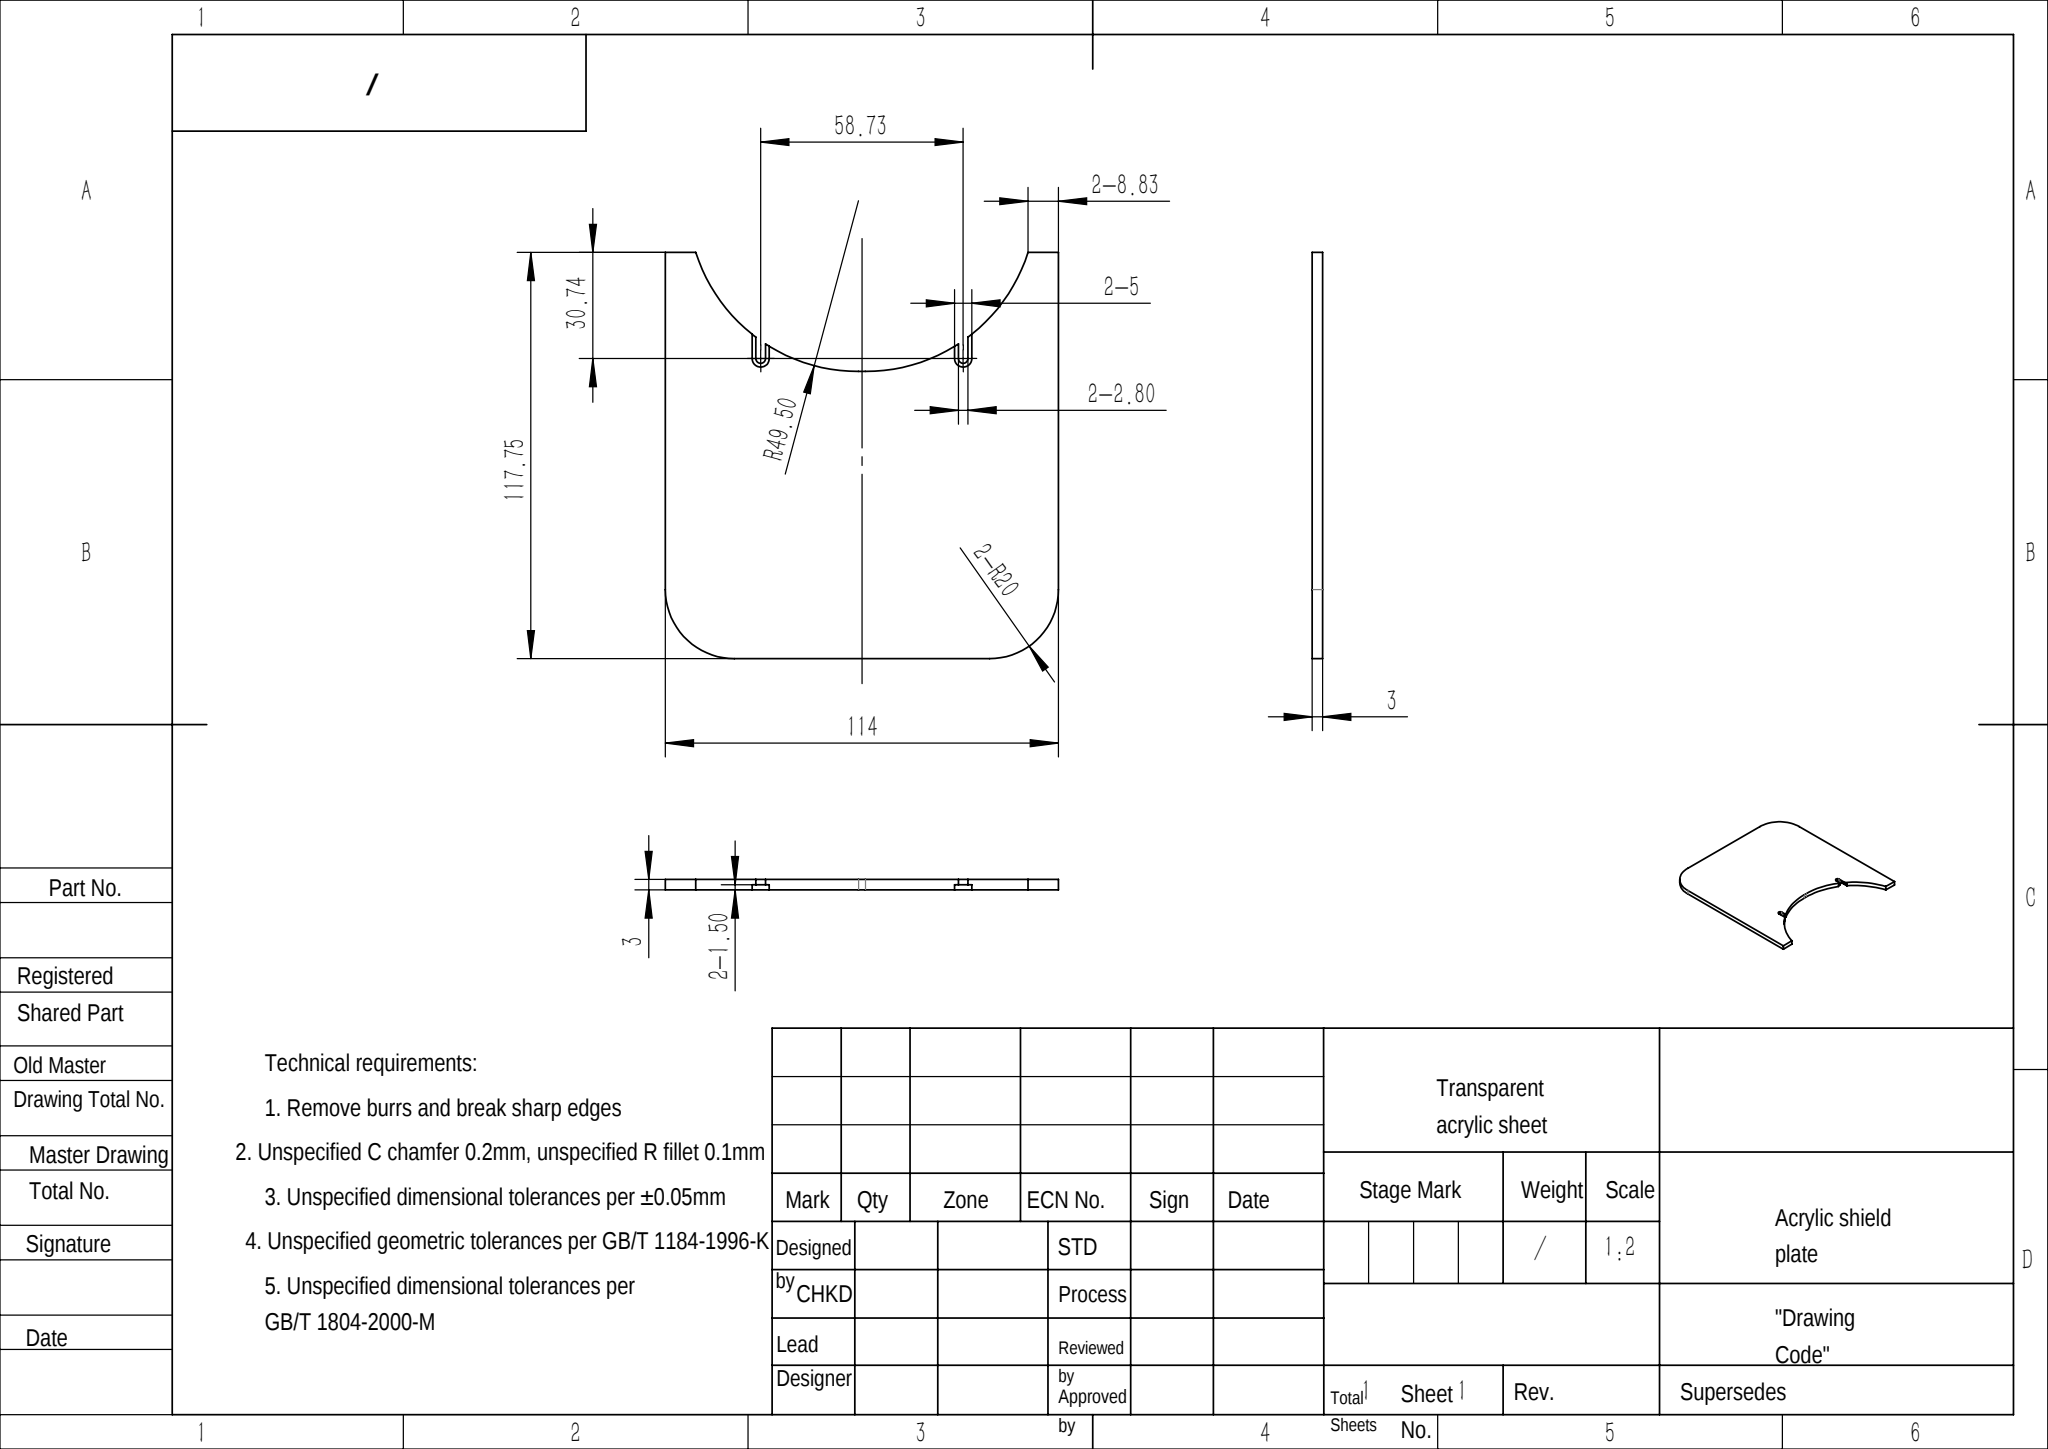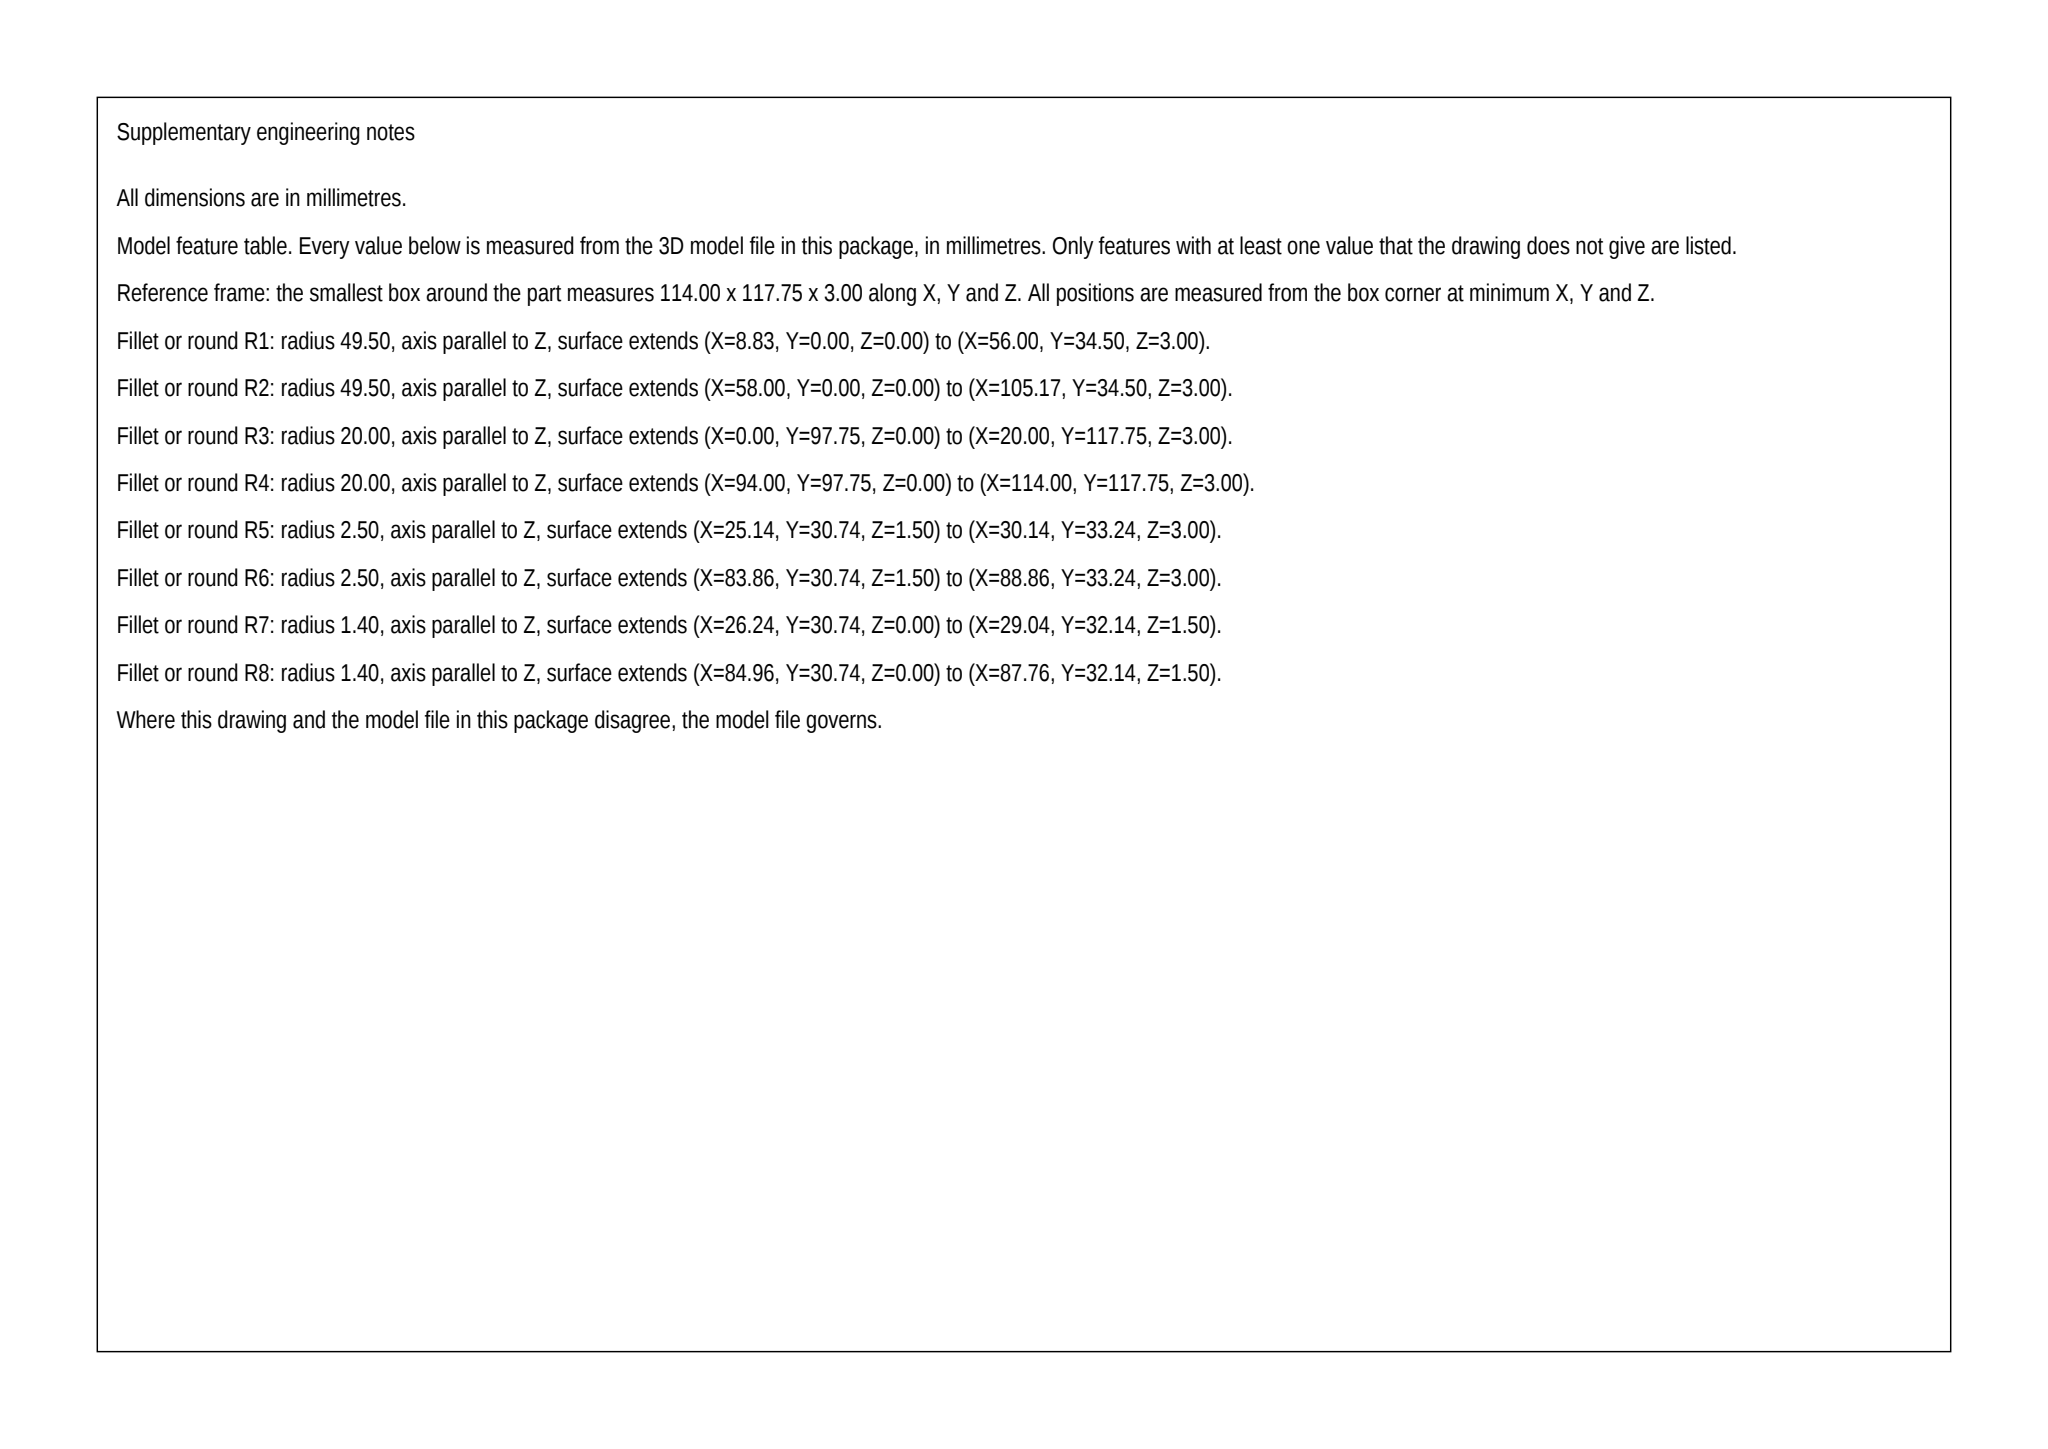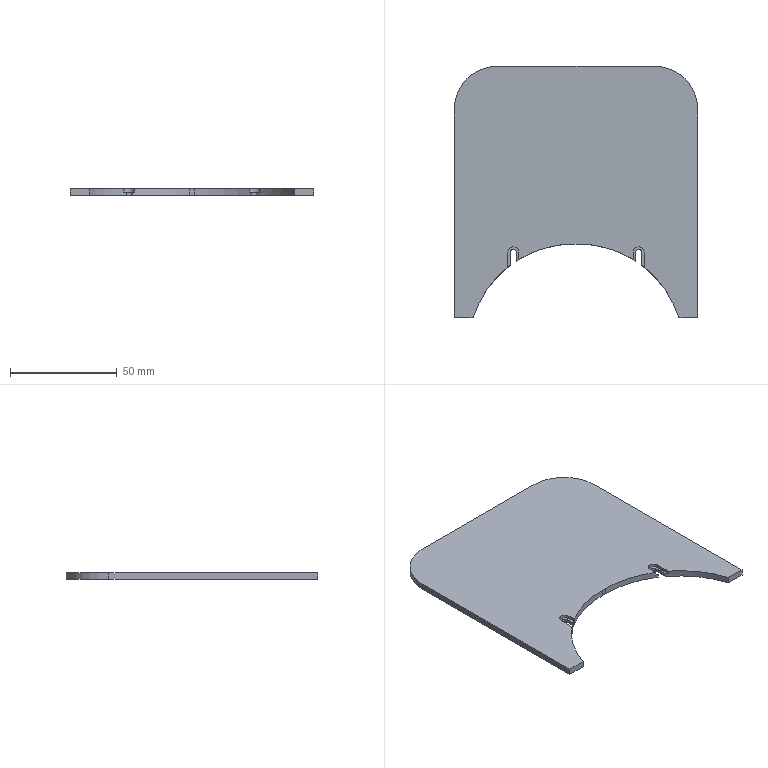Part | SolidWorks | mm | material Transparent acrylic sheet | 1 solid | 28 faces | box 114 x 117.75 x 3 mm | volume 32227 mm3 | plane 18 | cylinder 10 | commonest cylinder face diameters 99 x4 2.8 x2 40 x2 5 x2
STEP:
#1=CARTESIAN_POINT('',(27.964,141.858,1.5));
#2=VERTEX_POINT('',#1);
#3=CARTESIAN_POINT('',(30.764,141.858,1.5));
#4=VERTEX_POINT('',#3);
#5=CARTESIAN_POINT('',(29.364,141.858,1.5));
#6=DIRECTION('',(0.,0.,-1.));
#7=DIRECTION('',(1.,0.,0.));
#8=AXIS2_PLACEMENT_3D('',#5,#6,#7);
#9=CIRCLE('',#8,1.4);
#10=EDGE_CURVE('',#2,#4,#9,.T.);
#11=ORIENTED_EDGE('',*,*,#10,.F.);
#12=CARTESIAN_POINT('',(27.964,141.858,0.));
#13=VERTEX_POINT('',#12);
#14=CARTESIAN_POINT('',(27.964,141.858,-7.));
#15=DIRECTION('',(0.,0.,1.));
#16=VECTOR('',#15,1000.);
#17=LINE('',#14,#16);
#18=EDGE_CURVE('',#13,#2,#17,.T.);
#19=ORIENTED_EDGE('',*,*,#18,.F.);
#20=CARTESIAN_POINT('',(30.764,141.858,0.));
#21=VERTEX_POINT('',#20);
#22=CARTESIAN_POINT('',(29.364,141.858,0.));
#23=DIRECTION('',(0.,0.,1.));
#24=DIRECTION('',(1.,0.,0.));
#25=AXIS2_PLACEMENT_3D('',#22,#23,#24);
#26=CIRCLE('',#25,1.4);
#27=EDGE_CURVE('',#21,#13,#26,.T.);
#28=ORIENTED_EDGE('',*,*,#27,.F.);
#29=CARTESIAN_POINT('',(30.764,141.858,-7.));
#30=DIRECTION('',(0.,0.,1.));
#31=VECTOR('',#30,1000.);
#32=LINE('',#29,#31);
#33=EDGE_CURVE('',#21,#4,#32,.T.);
#34=ORIENTED_EDGE('',*,*,#33,.T.);
#35=EDGE_LOOP('',(#11,#19,#28,#34));
#36=FACE_OUTER_BOUND('',#35,.T.);
#37=CARTESIAN_POINT('',(29.364,141.858,-7.));
#38=DIRECTION('',(0.,0.,1.));
#39=DIRECTION('',(1.,0.,0.));
#40=AXIS2_PLACEMENT_3D('',#37,#38,#39);
#41=CYLINDRICAL_SURFACE('',#40,1.4);
#42=ADVANCED_FACE('',(#36),#41,.F.);
#43=CARTESIAN_POINT('',(30.764,135.668,1.5));
#44=VERTEX_POINT('',#43);
#45=CARTESIAN_POINT('',(30.764,132.725,1.5));
#46=DIRECTION('',(0.,-1.,0.));
#47=VECTOR('',#46,1000.);
#48=LINE('',#45,#47);
#49=EDGE_CURVE('',#4,#44,#48,.T.);
#50=ORIENTED_EDGE('',*,*,#49,.F.);
#51=ORIENTED_EDGE('',*,*,#33,.F.);
#52=CARTESIAN_POINT('',(30.764,135.668,0.));
#53=VERTEX_POINT('',#52);
#54=CARTESIAN_POINT('',(30.764,96.116,0.));
#55=DIRECTION('',(0.,1.,0.));
#56=VECTOR('',#55,1000.);
#57=LINE('',#54,#56);
#58=EDGE_CURVE('',#53,#21,#57,.T.);
#59=ORIENTED_EDGE('',*,*,#58,.F.);
#60=CARTESIAN_POINT('',(30.764,135.668,3.));
#61=DIRECTION('',(0.,0.,1.));
#62=VECTOR('',#61,1000.);
#63=LINE('',#60,#62);
#64=EDGE_CURVE('',#53,#44,#63,.T.);
#65=ORIENTED_EDGE('',*,*,#64,.T.);
#66=EDGE_LOOP('',(#50,#51,#59,#65));
#67=FACE_OUTER_BOUND('',#66,.T.);
#68=CARTESIAN_POINT('',(30.764,132.725,-7.));
#69=DIRECTION('',(1.,0.,0.));
#70=DIRECTION('',(0.,0.,-1.));
#71=AXIS2_PLACEMENT_3D('',#68,#69,#70);
#72=PLANE('',#71);
#73=ADVANCED_FACE('',(#67),#72,.F.);
#74=CARTESIAN_POINT('',(27.964,137.627,1.5));
#75=VERTEX_POINT('',#74);
#76=CARTESIAN_POINT('',(27.964,141.858,1.5));
#77=DIRECTION('',(0.,1.,0.));
#78=VECTOR('',#77,1000.);
#79=LINE('',#76,#78);
#80=EDGE_CURVE('',#75,#2,#79,.T.);
#81=ORIENTED_EDGE('',*,*,#80,.F.);
#82=CARTESIAN_POINT('',(27.964,137.627,0.));
#83=VERTEX_POINT('',#82);
#84=CARTESIAN_POINT('',(27.964,137.627,3.));
#85=DIRECTION('',(0.,0.,-1.));
#86=VECTOR('',#85,1000.);
#87=LINE('',#84,#86);
#88=EDGE_CURVE('',#75,#83,#87,.T.);
#89=ORIENTED_EDGE('',*,*,#88,.T.);
#90=CARTESIAN_POINT('',(27.964,96.116,0.));
#91=DIRECTION('',(0.,-1.,0.));
#92=VECTOR('',#91,1000.);
#93=LINE('',#90,#92);
#94=EDGE_CURVE('',#13,#83,#93,.T.);
#95=ORIENTED_EDGE('',*,*,#94,.F.);
#96=ORIENTED_EDGE('',*,*,#18,.T.);
#97=EDGE_LOOP('',(#81,#89,#95,#96));
#98=FACE_OUTER_BOUND('',#97,.T.);
#99=CARTESIAN_POINT('',(27.964,141.858,-7.));
#100=DIRECTION('',(-1.,0.,0.));
#101=DIRECTION('',(0.,0.,1.));
#102=AXIS2_PLACEMENT_3D('',#99,#100,#101);
#103=PLANE('',#102);
#104=ADVANCED_FACE('',(#98),#103,.F.);
#105=CARTESIAN_POINT('',(-30.764,141.858,1.5));
#106=VERTEX_POINT('',#105);
#107=CARTESIAN_POINT('',(-27.964,141.858,1.5));
#108=VERTEX_POINT('',#107);
#109=CARTESIAN_POINT('',(-29.364,141.858,1.5));
#110=DIRECTION('',(0.,0.,-1.));
#111=DIRECTION('',(1.,0.,0.));
#112=AXIS2_PLACEMENT_3D('',#109,#110,#111);
#113=CIRCLE('',#112,1.4);
#114=EDGE_CURVE('',#106,#108,#113,.T.);
#115=ORIENTED_EDGE('',*,*,#114,.F.);
#116=CARTESIAN_POINT('',(-30.764,141.858,0.));
#117=VERTEX_POINT('',#116);
#118=CARTESIAN_POINT('',(-30.764,141.858,-7.));
#119=DIRECTION('',(0.,0.,1.));
#120=VECTOR('',#119,1000.);
#121=LINE('',#118,#120);
#122=EDGE_CURVE('',#117,#106,#121,.T.);
#123=ORIENTED_EDGE('',*,*,#122,.F.);
#124=CARTESIAN_POINT('',(-27.964,141.858,0.));
#125=VERTEX_POINT('',#124);
#126=CARTESIAN_POINT('',(-29.364,141.858,0.));
#127=DIRECTION('',(0.,0.,1.));
#128=DIRECTION('',(1.,0.,0.));
#129=AXIS2_PLACEMENT_3D('',#126,#127,#128);
#130=CIRCLE('',#129,1.4);
#131=EDGE_CURVE('',#125,#117,#130,.T.);
#132=ORIENTED_EDGE('',*,*,#131,.F.);
#133=CARTESIAN_POINT('',(-27.964,141.858,-7.));
#134=DIRECTION('',(0.,0.,1.));
#135=VECTOR('',#134,1000.);
#136=LINE('',#133,#135);
#137=EDGE_CURVE('',#125,#108,#136,.T.);
#138=ORIENTED_EDGE('',*,*,#137,.T.);
#139=EDGE_LOOP('',(#115,#123,#132,#138));
#140=FACE_OUTER_BOUND('',#139,.T.);
#141=CARTESIAN_POINT('',(-29.364,141.858,-7.));
#142=DIRECTION('',(0.,0.,1.));
#143=DIRECTION('',(1.,0.,0.));
#144=AXIS2_PLACEMENT_3D('',#141,#142,#143);
#145=CYLINDRICAL_SURFACE('',#144,1.4);
#146=ADVANCED_FACE('',(#140),#145,.F.);
#147=CARTESIAN_POINT('',(-27.964,137.627,1.5));
#148=VERTEX_POINT('',#147);
#149=CARTESIAN_POINT('',(-27.964,131.981,1.5));
#150=DIRECTION('',(0.,-1.,0.));
#151=VECTOR('',#150,1000.);
#152=LINE('',#149,#151);
#153=EDGE_CURVE('',#108,#148,#152,.T.);
#154=ORIENTED_EDGE('',*,*,#153,.F.);
#155=ORIENTED_EDGE('',*,*,#137,.F.);
#156=CARTESIAN_POINT('',(-27.964,137.627,0.));
#157=VERTEX_POINT('',#156);
#158=CARTESIAN_POINT('',(-27.964,96.116,0.));
#159=DIRECTION('',(0.,1.,0.));
#160=VECTOR('',#159,1000.);
#161=LINE('',#158,#160);
#162=EDGE_CURVE('',#157,#125,#161,.T.);
#163=ORIENTED_EDGE('',*,*,#162,.F.);
#164=CARTESIAN_POINT('',(-27.964,137.627,3.));
#165=DIRECTION('',(0.,0.,1.));
#166=VECTOR('',#165,1000.);
#167=LINE('',#164,#166);
#168=EDGE_CURVE('',#157,#148,#167,.T.);
#169=ORIENTED_EDGE('',*,*,#168,.T.);
#170=EDGE_LOOP('',(#154,#155,#163,#169));
#171=FACE_OUTER_BOUND('',#170,.T.);
#172=CARTESIAN_POINT('',(-27.964,131.981,-7.));
#173=DIRECTION('',(1.,0.,0.));
#174=DIRECTION('',(0.,0.,-1.));
#175=AXIS2_PLACEMENT_3D('',#172,#173,#174);
#176=PLANE('',#175);
#177=ADVANCED_FACE('',(#171),#176,.F.);
#178=CARTESIAN_POINT('',(-30.764,135.668,1.5));
#179=VERTEX_POINT('',#178);
#180=CARTESIAN_POINT('',(-30.764,141.858,1.5));
#181=DIRECTION('',(0.,1.,0.));
#182=VECTOR('',#181,1000.);
#183=LINE('',#180,#182);
#184=EDGE_CURVE('',#179,#106,#183,.T.);
#185=ORIENTED_EDGE('',*,*,#184,.F.);
#186=CARTESIAN_POINT('',(-30.764,135.668,0.));
#187=VERTEX_POINT('',#186);
#188=CARTESIAN_POINT('',(-30.764,135.668,3.));
#189=DIRECTION('',(0.,0.,-1.));
#190=VECTOR('',#189,1000.);
#191=LINE('',#188,#190);
#192=EDGE_CURVE('',#179,#187,#191,.T.);
#193=ORIENTED_EDGE('',*,*,#192,.T.);
#194=CARTESIAN_POINT('',(-30.764,96.116,0.));
#195=DIRECTION('',(0.,-1.,0.));
#196=VECTOR('',#195,1000.);
#197=LINE('',#194,#196);
#198=EDGE_CURVE('',#117,#187,#197,.T.);
#199=ORIENTED_EDGE('',*,*,#198,.F.);
#200=ORIENTED_EDGE('',*,*,#122,.T.);
#201=EDGE_LOOP('',(#185,#193,#199,#200));
#202=FACE_OUTER_BOUND('',#201,.T.);
#203=CARTESIAN_POINT('',(-30.764,141.858,-7.));
#204=DIRECTION('',(-1.,0.,0.));
#205=DIRECTION('',(0.,0.,1.));
#206=AXIS2_PLACEMENT_3D('',#203,#204,#205);
#207=PLANE('',#206);
#208=ADVANCED_FACE('',(#202),#207,.F.);
#209=CARTESIAN_POINT('',(31.864,134.816,1.5));
#210=VERTEX_POINT('',#209);
#211=CARTESIAN_POINT('',(31.864,134.816,3.));
#212=VERTEX_POINT('',#211);
#213=CARTESIAN_POINT('',(31.864,134.816,3.));
#214=DIRECTION('',(0.,0.,1.));
#215=VECTOR('',#214,1000.);
#216=LINE('',#213,#215);
#217=EDGE_CURVE('',#210,#212,#216,.T.);
#218=ORIENTED_EDGE('',*,*,#217,.F.);
#219=CARTESIAN_POINT('',(1.,96.116,1.5));
#220=DIRECTION('',(0.,0.,1.));
#221=DIRECTION('',(1.,0.,0.));
#222=AXIS2_PLACEMENT_3D('',#219,#220,#221);
#223=CIRCLE('',#222,49.5);
#224=EDGE_CURVE('',#210,#44,#223,.T.);
#225=ORIENTED_EDGE('',*,*,#224,.T.);
#226=ORIENTED_EDGE('',*,*,#64,.F.);
#227=CARTESIAN_POINT('',(48.173,111.116,0.));
#228=VERTEX_POINT('',#227);
#229=CARTESIAN_POINT('',(1.,96.116,0.));
#230=DIRECTION('',(0.,0.,1.));
#231=DIRECTION('',(1.,0.,0.));
#232=AXIS2_PLACEMENT_3D('',#229,#230,#231);
#233=CIRCLE('',#232,49.5);
#234=EDGE_CURVE('',#228,#53,#233,.T.);
#235=ORIENTED_EDGE('',*,*,#234,.F.);
#236=CARTESIAN_POINT('',(48.173,111.116,3.));
#237=VERTEX_POINT('',#236);
#238=CARTESIAN_POINT('',(48.173,111.116,3.));
#239=DIRECTION('',(0.,0.,-1.));
#240=VECTOR('',#239,1000.);
#241=LINE('',#238,#240);
#242=EDGE_CURVE('',#237,#228,#241,.T.);
#243=ORIENTED_EDGE('',*,*,#242,.F.);
#244=CARTESIAN_POINT('',(1.,96.116,3.));
#245=DIRECTION('',(0.,0.,1.));
#246=DIRECTION('',(1.,0.,0.));
#247=AXIS2_PLACEMENT_3D('',#244,#245,#246);
#248=CIRCLE('',#247,49.5);
#249=EDGE_CURVE('',#237,#212,#248,.T.);
#250=ORIENTED_EDGE('',*,*,#249,.T.);
#251=EDGE_LOOP('',(#218,#225,#226,#235,#243,#250));
#252=FACE_OUTER_BOUND('',#251,.T.);
#253=CARTESIAN_POINT('',(1.,96.116,3.));
#254=DIRECTION('',(0.,0.,-1.));
#255=DIRECTION('',(-1.,0.,0.));
#256=AXIS2_PLACEMENT_3D('',#253,#254,#255);
#257=CYLINDRICAL_SURFACE('',#256,49.5);
#258=ADVANCED_FACE('',(#252),#257,.F.);
#259=CARTESIAN_POINT('',(-26.864,138.321,1.5));
#260=VERTEX_POINT('',#259);
#261=CARTESIAN_POINT('',(-26.864,138.321,3.));
#262=VERTEX_POINT('',#261);
#263=CARTESIAN_POINT('',(-26.864,138.321,3.));
#264=DIRECTION('',(0.,0.,1.));
#265=VECTOR('',#264,1000.);
#266=LINE('',#263,#265);
#267=EDGE_CURVE('',#260,#262,#266,.T.);
#268=ORIENTED_EDGE('',*,*,#267,.F.);
#269=CARTESIAN_POINT('',(-1.,96.116,1.5));
#270=DIRECTION('',(0.,0.,1.));
#271=DIRECTION('',(1.,0.,0.));
#272=AXIS2_PLACEMENT_3D('',#269,#270,#271);
#273=CIRCLE('',#272,49.5);
#274=EDGE_CURVE('',#260,#148,#273,.T.);
#275=ORIENTED_EDGE('',*,*,#274,.T.);
#276=ORIENTED_EDGE('',*,*,#168,.F.);
#277=CARTESIAN_POINT('',(-1.,145.616,0.));
#278=VERTEX_POINT('',#277);
#279=CARTESIAN_POINT('',(-1.,96.116,0.));
#280=DIRECTION('',(0.,0.,1.));
#281=DIRECTION('',(1.,0.,0.));
#282=AXIS2_PLACEMENT_3D('',#279,#280,#281);
#283=CIRCLE('',#282,49.5);
#284=EDGE_CURVE('',#278,#157,#283,.T.);
#285=ORIENTED_EDGE('',*,*,#284,.F.);
#286=CARTESIAN_POINT('',(-1.,145.616,3.));
#287=VERTEX_POINT('',#286);
#288=CARTESIAN_POINT('',(-1.,145.616,3.));
#289=DIRECTION('',(0.,0.,-1.));
#290=VECTOR('',#289,1000.);
#291=LINE('',#288,#290);
#292=EDGE_CURVE('',#287,#278,#291,.T.);
#293=ORIENTED_EDGE('',*,*,#292,.F.);
#294=CARTESIAN_POINT('',(-1.,96.116,3.));
#295=DIRECTION('',(0.,0.,1.));
#296=DIRECTION('',(1.,0.,0.));
#297=AXIS2_PLACEMENT_3D('',#294,#295,#296);
#298=CIRCLE('',#297,49.5);
#299=EDGE_CURVE('',#287,#262,#298,.T.);
#300=ORIENTED_EDGE('',*,*,#299,.T.);
#301=EDGE_LOOP('',(#268,#275,#276,#285,#293,#300));
#302=FACE_OUTER_BOUND('',#301,.T.);
#303=CARTESIAN_POINT('',(-1.,96.116,3.));
#304=DIRECTION('',(0.,0.,-1.));
#305=DIRECTION('',(-1.,0.,0.));
#306=AXIS2_PLACEMENT_3D('',#303,#304,#305);
#307=CYLINDRICAL_SURFACE('',#306,49.5);
#308=ADVANCED_FACE('',(#302),#307,.F.);
#309=CARTESIAN_POINT('',(1.,145.616,0.));
#310=VERTEX_POINT('',#309);
#311=CARTESIAN_POINT('',(-1.,145.616,0.));
#312=DIRECTION('',(1.,0.,0.));
#313=VECTOR('',#312,1000.);
#314=LINE('',#311,#313);
#315=EDGE_CURVE('',#278,#310,#314,.T.);
#316=ORIENTED_EDGE('',*,*,#315,.T.);
#317=CARTESIAN_POINT('',(1.,145.616,3.));
#318=VERTEX_POINT('',#317);
#319=CARTESIAN_POINT('',(1.,145.616,3.));
#320=DIRECTION('',(0.,0.,-1.));
#321=VECTOR('',#320,1000.);
#322=LINE('',#319,#321);
#323=EDGE_CURVE('',#318,#310,#322,.T.);
#324=ORIENTED_EDGE('',*,*,#323,.F.);
#325=CARTESIAN_POINT('',(-1.,145.616,3.));
#326=DIRECTION('',(1.,0.,0.));
#327=VECTOR('',#326,1000.);
#328=LINE('',#325,#327);
#329=EDGE_CURVE('',#287,#318,#328,.T.);
#330=ORIENTED_EDGE('',*,*,#329,.F.);
#331=ORIENTED_EDGE('',*,*,#292,.T.);
#332=EDGE_LOOP('',(#316,#324,#330,#331));
#333=FACE_OUTER_BOUND('',#332,.T.);
#334=CARTESIAN_POINT('',(-1.,145.616,3.));
#335=DIRECTION('',(0.,1.,0.));
#336=DIRECTION('',(0.,0.,1.));
#337=AXIS2_PLACEMENT_3D('',#334,#335,#336);
#338=PLANE('',#337);
#339=ADVANCED_FACE('',(#333),#338,.F.);
#340=CARTESIAN_POINT('',(26.864,138.321,3.));
#341=VERTEX_POINT('',#340);
#342=CARTESIAN_POINT('',(26.864,138.321,1.5));
#343=VERTEX_POINT('',#342);
#344=CARTESIAN_POINT('',(26.864,138.321,3.));
#345=DIRECTION('',(0.,0.,-1.));
#346=VECTOR('',#345,1000.);
#347=LINE('',#344,#346);
#348=EDGE_CURVE('',#341,#343,#347,.T.);
#349=ORIENTED_EDGE('',*,*,#348,.F.);
#350=CARTESIAN_POINT('',(1.,96.116,3.));
#351=DIRECTION('',(0.,0.,1.));
#352=DIRECTION('',(1.,0.,0.));
#353=AXIS2_PLACEMENT_3D('',#350,#351,#352);
#354=CIRCLE('',#353,49.5);
#355=EDGE_CURVE('',#341,#318,#354,.T.);
#356=ORIENTED_EDGE('',*,*,#355,.T.);
#357=ORIENTED_EDGE('',*,*,#323,.T.);
#358=CARTESIAN_POINT('',(1.,96.116,0.));
#359=DIRECTION('',(0.,0.,1.));
#360=DIRECTION('',(1.,0.,0.));
#361=AXIS2_PLACEMENT_3D('',#358,#359,#360);
#362=CIRCLE('',#361,49.5);
#363=EDGE_CURVE('',#83,#310,#362,.T.);
#364=ORIENTED_EDGE('',*,*,#363,.F.);
#365=ORIENTED_EDGE('',*,*,#88,.F.);
#366=CARTESIAN_POINT('',(1.,96.116,1.5));
#367=DIRECTION('',(0.,0.,1.));
#368=DIRECTION('',(1.,0.,0.));
#369=AXIS2_PLACEMENT_3D('',#366,#367,#368);
#370=CIRCLE('',#369,49.5);
#371=EDGE_CURVE('',#75,#343,#370,.T.);
#372=ORIENTED_EDGE('',*,*,#371,.T.);
#373=EDGE_LOOP('',(#349,#356,#357,#364,#365,#372));
#374=FACE_OUTER_BOUND('',#373,.T.);
#375=CARTESIAN_POINT('',(1.,96.116,3.));
#376=DIRECTION('',(0.,0.,-1.));
#377=DIRECTION('',(-1.,0.,0.));
#378=AXIS2_PLACEMENT_3D('',#375,#376,#377);
#379=CYLINDRICAL_SURFACE('',#378,49.5);
#380=ADVANCED_FACE('',(#374),#379,.F.);
#381=CARTESIAN_POINT('',(57.,111.116,0.));
#382=VERTEX_POINT('',#381);
#383=CARTESIAN_POINT('',(56.,111.116,0.));
#384=DIRECTION('',(1.,0.,0.));
#385=VECTOR('',#384,1000.);
#386=LINE('',#383,#385);
#387=EDGE_CURVE('',#228,#382,#386,.T.);
#388=ORIENTED_EDGE('',*,*,#387,.T.);
#389=CARTESIAN_POINT('',(57.,111.116,3.));
#390=VERTEX_POINT('',#389);
#391=CARTESIAN_POINT('',(57.,111.116,3.));
#392=DIRECTION('',(0.,0.,-1.));
#393=VECTOR('',#392,1000.);
#394=LINE('',#391,#393);
#395=EDGE_CURVE('',#390,#382,#394,.T.);
#396=ORIENTED_EDGE('',*,*,#395,.F.);
#397=CARTESIAN_POINT('',(56.,111.116,3.));
#398=DIRECTION('',(1.,0.,0.));
#399=VECTOR('',#398,1000.);
#400=LINE('',#397,#399);
#401=EDGE_CURVE('',#237,#390,#400,.T.);
#402=ORIENTED_EDGE('',*,*,#401,.F.);
#403=ORIENTED_EDGE('',*,*,#242,.T.);
#404=EDGE_LOOP('',(#388,#396,#402,#403));
#405=FACE_OUTER_BOUND('',#404,.T.);
#406=CARTESIAN_POINT('',(56.,111.116,3.));
#407=DIRECTION('',(0.,1.,0.));
#408=DIRECTION('',(0.,0.,1.));
#409=AXIS2_PLACEMENT_3D('',#406,#407,#408);
#410=PLANE('',#409);
#411=ADVANCED_FACE('',(#405),#410,.F.);
#412=CARTESIAN_POINT('',(57.,208.864,0.));
#413=VERTEX_POINT('',#412);
#414=CARTESIAN_POINT('',(57.,96.116,0.));
#415=DIRECTION('',(-0.,1.,0.));
#416=VECTOR('',#415,1000.);
#417=LINE('',#414,#416);
#418=EDGE_CURVE('',#382,#413,#417,.T.);
#419=ORIENTED_EDGE('',*,*,#418,.T.);
#420=CARTESIAN_POINT('',(57.,208.864,3.));
#421=VERTEX_POINT('',#420);
#422=CARTESIAN_POINT('',(57.,208.864,3.));
#423=DIRECTION('',(0.,0.,1.));
#424=VECTOR('',#423,1000.);
#425=LINE('',#422,#424);
#426=EDGE_CURVE('',#413,#421,#425,.T.);
#427=ORIENTED_EDGE('',*,*,#426,.T.);
#428=CARTESIAN_POINT('',(57.,96.116,3.));
#429=DIRECTION('',(-0.,1.,0.));
#430=VECTOR('',#429,1000.);
#431=LINE('',#428,#430);
#432=EDGE_CURVE('',#390,#421,#431,.T.);
#433=ORIENTED_EDGE('',*,*,#432,.F.);
#434=ORIENTED_EDGE('',*,*,#395,.T.);
#435=EDGE_LOOP('',(#419,#427,#433,#434));
#436=FACE_OUTER_BOUND('',#435,.T.);
#437=CARTESIAN_POINT('',(57.,96.116,3.));
#438=DIRECTION('',(-1.,-0.,0.));
#439=DIRECTION('',(0.,-1.,0.));
#440=AXIS2_PLACEMENT_3D('',#437,#438,#439);
#441=PLANE('',#440);
#442=ADVANCED_FACE('',(#436),#441,.F.);
#443=CARTESIAN_POINT('',(-37.,228.864,0.));
#444=VERTEX_POINT('',#443);
#445=CARTESIAN_POINT('',(37.,228.864,0.));
#446=VERTEX_POINT('',#445);
#447=CARTESIAN_POINT('',(-60.,228.864,0.));
#448=DIRECTION('',(1.,0.,0.));
#449=VECTOR('',#448,1000.);
#450=LINE('',#447,#449);
#451=EDGE_CURVE('',#444,#446,#450,.T.);
#452=ORIENTED_EDGE('',*,*,#451,.F.);
#453=CARTESIAN_POINT('',(-37.,228.864,3.));
#454=VERTEX_POINT('',#453);
#455=CARTESIAN_POINT('',(-37.,228.864,3.));
#456=DIRECTION('',(0.,0.,1.));
#457=VECTOR('',#456,1000.);
#458=LINE('',#455,#457);
#459=EDGE_CURVE('',#444,#454,#458,.T.);
#460=ORIENTED_EDGE('',*,*,#459,.T.);
#461=CARTESIAN_POINT('',(37.,228.864,3.));
#462=VERTEX_POINT('',#461);
#463=CARTESIAN_POINT('',(-60.,228.864,3.));
#464=DIRECTION('',(1.,0.,0.));
#465=VECTOR('',#464,1000.);
#466=LINE('',#463,#465);
#467=EDGE_CURVE('',#454,#462,#466,.T.);
#468=ORIENTED_EDGE('',*,*,#467,.T.);
#469=CARTESIAN_POINT('',(37.,228.864,0.));
#470=DIRECTION('',(0.,0.,-1.));
#471=VECTOR('',#470,1000.);
#472=LINE('',#469,#471);
#473=EDGE_CURVE('',#462,#446,#472,.T.);
#474=ORIENTED_EDGE('',*,*,#473,.T.);
#475=EDGE_LOOP('',(#452,#460,#468,#474));
#476=FACE_OUTER_BOUND('',#475,.T.);
#477=CARTESIAN_POINT('',(-60.,228.864,3.));
#478=DIRECTION('',(-0.,1.,0.));
#479=DIRECTION('',(-1.,-0.,0.));
#480=AXIS2_PLACEMENT_3D('',#477,#478,#479);
#481=PLANE('',#480);
#482=ADVANCED_FACE('',(#476),#481,.T.);
#483=CARTESIAN_POINT('',(-57.,111.116,3.));
#484=VERTEX_POINT('',#483);
#485=CARTESIAN_POINT('',(-57.,208.864,3.));
#486=VERTEX_POINT('',#485);
#487=CARTESIAN_POINT('',(-57.,96.116,3.));
#488=DIRECTION('',(0.,1.,0.));
#489=VECTOR('',#488,1000.);
#490=LINE('',#487,#489);
#491=EDGE_CURVE('',#484,#486,#490,.T.);
#492=ORIENTED_EDGE('',*,*,#491,.T.);
#493=CARTESIAN_POINT('',(-57.,208.864,0.));
#494=VERTEX_POINT('',#493);
#495=CARTESIAN_POINT('',(-57.,208.864,3.));
#496=DIRECTION('',(0.,0.,-1.));
#497=VECTOR('',#496,1000.);
#498=LINE('',#495,#497);
#499=EDGE_CURVE('',#486,#494,#498,.T.);
#500=ORIENTED_EDGE('',*,*,#499,.T.);
#501=CARTESIAN_POINT('',(-57.,111.116,0.));
#502=VERTEX_POINT('',#501);
#503=CARTESIAN_POINT('',(-57.,96.116,0.));
#504=DIRECTION('',(0.,1.,0.));
#505=VECTOR('',#504,1000.);
#506=LINE('',#503,#505);
#507=EDGE_CURVE('',#502,#494,#506,.T.);
#508=ORIENTED_EDGE('',*,*,#507,.F.);
#509=CARTESIAN_POINT('',(-57.,111.116,3.));
#510=DIRECTION('',(0.,0.,-1.));
#511=VECTOR('',#510,1000.);
#512=LINE('',#509,#511);
#513=EDGE_CURVE('',#484,#502,#512,.T.);
#514=ORIENTED_EDGE('',*,*,#513,.F.);
#515=EDGE_LOOP('',(#492,#500,#508,#514));
#516=FACE_OUTER_BOUND('',#515,.T.);
#517=CARTESIAN_POINT('',(-57.,96.116,3.));
#518=DIRECTION('',(-1.,0.,0.));
#519=DIRECTION('',(0.,0.,1.));
#520=AXIS2_PLACEMENT_3D('',#517,#518,#519);
#521=PLANE('',#520);
#522=ADVANCED_FACE('',(#516),#521,.T.);
#523=CARTESIAN_POINT('',(-48.173,111.116,0.));
#524=VERTEX_POINT('',#523);
#525=CARTESIAN_POINT('',(-60.,111.116,0.));
#526=DIRECTION('',(1.,0.,0.));
#527=VECTOR('',#526,1000.);
#528=LINE('',#525,#527);
#529=EDGE_CURVE('',#502,#524,#528,.T.);
#530=ORIENTED_EDGE('',*,*,#529,.T.);
#531=CARTESIAN_POINT('',(-48.173,111.116,3.));
#532=VERTEX_POINT('',#531);
#533=CARTESIAN_POINT('',(-48.173,111.116,3.));
#534=DIRECTION('',(0.,0.,-1.));
#535=VECTOR('',#534,1000.);
#536=LINE('',#533,#535);
#537=EDGE_CURVE('',#532,#524,#536,.T.);
#538=ORIENTED_EDGE('',*,*,#537,.F.);
#539=CARTESIAN_POINT('',(-60.,111.116,3.));
#540=DIRECTION('',(1.,0.,0.));
#541=VECTOR('',#540,1000.);
#542=LINE('',#539,#541);
#543=EDGE_CURVE('',#484,#532,#542,.T.);
#544=ORIENTED_EDGE('',*,*,#543,.F.);
#545=ORIENTED_EDGE('',*,*,#513,.T.);
#546=EDGE_LOOP('',(#530,#538,#544,#545));
#547=FACE_OUTER_BOUND('',#546,.T.);
#548=CARTESIAN_POINT('',(-60.,111.116,3.));
#549=DIRECTION('',(0.,1.,0.));
#550=DIRECTION('',(0.,0.,1.));
#551=AXIS2_PLACEMENT_3D('',#548,#549,#550);
#552=PLANE('',#551);
#553=ADVANCED_FACE('',(#547),#552,.F.);
#554=CARTESIAN_POINT('',(-31.864,134.816,3.));
#555=VERTEX_POINT('',#554);
#556=CARTESIAN_POINT('',(-31.864,134.816,1.5));
#557=VERTEX_POINT('',#556);
#558=CARTESIAN_POINT('',(-31.864,134.816,3.));
#559=DIRECTION('',(0.,0.,-1.));
#560=VECTOR('',#559,1000.);
#561=LINE('',#558,#560);
#562=EDGE_CURVE('',#555,#557,#561,.T.);
#563=ORIENTED_EDGE('',*,*,#562,.F.);
#564=CARTESIAN_POINT('',(-1.,96.116,3.));
#565=DIRECTION('',(0.,0.,1.));
#566=DIRECTION('',(1.,0.,0.));
#567=AXIS2_PLACEMENT_3D('',#564,#565,#566);
#568=CIRCLE('',#567,49.5);
#569=EDGE_CURVE('',#555,#532,#568,.T.);
#570=ORIENTED_EDGE('',*,*,#569,.T.);
#571=ORIENTED_EDGE('',*,*,#537,.T.);
#572=CARTESIAN_POINT('',(-1.,96.116,0.));
#573=DIRECTION('',(0.,0.,1.));
#574=DIRECTION('',(1.,0.,0.));
#575=AXIS2_PLACEMENT_3D('',#572,#573,#574);
#576=CIRCLE('',#575,49.5);
#577=EDGE_CURVE('',#187,#524,#576,.T.);
#578=ORIENTED_EDGE('',*,*,#577,.F.);
#579=ORIENTED_EDGE('',*,*,#192,.F.);
#580=CARTESIAN_POINT('',(-1.,96.116,1.5));
#581=DIRECTION('',(0.,0.,1.));
#582=DIRECTION('',(1.,0.,0.));
#583=AXIS2_PLACEMENT_3D('',#580,#581,#582);
#584=CIRCLE('',#583,49.5);
#585=EDGE_CURVE('',#179,#557,#584,.T.);
#586=ORIENTED_EDGE('',*,*,#585,.T.);
#587=EDGE_LOOP('',(#563,#570,#571,#578,#579,#586));
#588=FACE_OUTER_BOUND('',#587,.T.);
#589=CARTESIAN_POINT('',(-1.,96.116,3.));
#590=DIRECTION('',(0.,0.,-1.));
#591=DIRECTION('',(-1.,0.,0.));
#592=AXIS2_PLACEMENT_3D('',#589,#590,#591);
#593=CYLINDRICAL_SURFACE('',#592,49.5);
#594=ADVANCED_FACE('',(#588),#593,.F.);
#595=CARTESIAN_POINT('',(-26.864,141.858,3.));
#596=VERTEX_POINT('',#595);
#597=CARTESIAN_POINT('',(-26.864,129.167,3.));
#598=DIRECTION('',(0.,1.,0.));
#599=VECTOR('',#598,1000.);
#600=LINE('',#597,#599);
#601=EDGE_CURVE('',#262,#596,#600,.T.);
#602=ORIENTED_EDGE('',*,*,#601,.F.);
#603=ORIENTED_EDGE('',*,*,#299,.F.);
#604=ORIENTED_EDGE('',*,*,#329,.T.);
#605=ORIENTED_EDGE('',*,*,#355,.F.);
#606=CARTESIAN_POINT('',(26.864,141.858,3.));
#607=VERTEX_POINT('',#606);
#608=CARTESIAN_POINT('',(26.864,141.858,3.));
#609=DIRECTION('',(0.,-1.,0.));
#610=VECTOR('',#609,1000.);
#611=LINE('',#608,#610);
#612=EDGE_CURVE('',#607,#341,#611,.T.);
#613=ORIENTED_EDGE('',*,*,#612,.F.);
#614=CARTESIAN_POINT('',(31.864,141.858,3.));
#615=VERTEX_POINT('',#614);
#616=CARTESIAN_POINT('',(29.364,141.858,3.));
#617=DIRECTION('',(0.,0.,1.));
#618=DIRECTION('',(1.,0.,0.));
#619=AXIS2_PLACEMENT_3D('',#616,#617,#618);
#620=CIRCLE('',#619,2.5);
#621=EDGE_CURVE('',#615,#607,#620,.T.);
#622=ORIENTED_EDGE('',*,*,#621,.F.);
#623=CARTESIAN_POINT('',(31.864,128.101,3.));
#624=DIRECTION('',(0.,1.,0.));
#625=VECTOR('',#624,1000.);
#626=LINE('',#623,#625);
#627=EDGE_CURVE('',#212,#615,#626,.T.);
#628=ORIENTED_EDGE('',*,*,#627,.F.);
#629=ORIENTED_EDGE('',*,*,#249,.F.);
#630=ORIENTED_EDGE('',*,*,#401,.T.);
#631=ORIENTED_EDGE('',*,*,#432,.T.);
#632=CARTESIAN_POINT('',(37.,208.864,3.));
#633=DIRECTION('',(0.,0.,1.));
#634=DIRECTION('',(1.,0.,0.));
#635=AXIS2_PLACEMENT_3D('',#632,#633,#634);
#636=CIRCLE('',#635,20.);
#637=EDGE_CURVE('',#421,#462,#636,.T.);
#638=ORIENTED_EDGE('',*,*,#637,.T.);
#639=ORIENTED_EDGE('',*,*,#467,.F.);
#640=CARTESIAN_POINT('',(-37.,208.864,3.));
#641=DIRECTION('',(0.,0.,1.));
#642=DIRECTION('',(1.,0.,0.));
#643=AXIS2_PLACEMENT_3D('',#640,#641,#642);
#644=CIRCLE('',#643,20.);
#645=EDGE_CURVE('',#454,#486,#644,.T.);
#646=ORIENTED_EDGE('',*,*,#645,.T.);
#647=ORIENTED_EDGE('',*,*,#491,.F.);
#648=ORIENTED_EDGE('',*,*,#543,.T.);
#649=ORIENTED_EDGE('',*,*,#569,.F.);
#650=CARTESIAN_POINT('',(-31.864,141.858,3.));
#651=VERTEX_POINT('',#650);
#652=CARTESIAN_POINT('',(-31.864,141.858,3.));
#653=DIRECTION('',(0.,-1.,0.));
#654=VECTOR('',#653,1000.);
#655=LINE('',#652,#654);
#656=EDGE_CURVE('',#651,#555,#655,.T.);
#657=ORIENTED_EDGE('',*,*,#656,.F.);
#658=CARTESIAN_POINT('',(-29.364,141.858,3.));
#659=DIRECTION('',(0.,0.,1.));
#660=DIRECTION('',(1.,0.,0.));
#661=AXIS2_PLACEMENT_3D('',#658,#659,#660);
#662=CIRCLE('',#661,2.5);
#663=EDGE_CURVE('',#596,#651,#662,.T.);
#664=ORIENTED_EDGE('',*,*,#663,.F.);
#665=EDGE_LOOP('',(#602,#603,#604,#605,#613,#622,#628,#629,#630,#631,#638,#639,#646,#647,#648,#649,#657,#664));
#666=FACE_OUTER_BOUND('',#665,.T.);
#667=CARTESIAN_POINT('',(1.,96.116,3.));
#668=DIRECTION('',(0.,0.,1.));
#669=DIRECTION('',(1.,0.,0.));
#670=AXIS2_PLACEMENT_3D('',#667,#668,#669);
#671=PLANE('',#670);
#672=ADVANCED_FACE('',(#666),#671,.T.);
#673=ORIENTED_EDGE('',*,*,#284,.T.);
#674=ORIENTED_EDGE('',*,*,#162,.T.);
#675=ORIENTED_EDGE('',*,*,#131,.T.);
#676=ORIENTED_EDGE('',*,*,#198,.T.);
#677=ORIENTED_EDGE('',*,*,#577,.T.);
#678=ORIENTED_EDGE('',*,*,#529,.F.);
#679=ORIENTED_EDGE('',*,*,#507,.T.);
#680=CARTESIAN_POINT('',(-37.,208.864,0.));
#681=DIRECTION('',(0.,0.,-1.));
#682=DIRECTION('',(1.,-0.,0.));
#683=AXIS2_PLACEMENT_3D('',#680,#681,#682);
#684=CIRCLE('',#683,20.);
#685=EDGE_CURVE('',#494,#444,#684,.T.);
#686=ORIENTED_EDGE('',*,*,#685,.T.);
#687=ORIENTED_EDGE('',*,*,#451,.T.);
#688=CARTESIAN_POINT('',(37.,208.864,0.));
#689=DIRECTION('',(0.,0.,-1.));
#690=DIRECTION('',(1.,0.,0.));
#691=AXIS2_PLACEMENT_3D('',#688,#689,#690);
#692=CIRCLE('',#691,20.);
#693=EDGE_CURVE('',#446,#413,#692,.T.);
#694=ORIENTED_EDGE('',*,*,#693,.T.);
#695=ORIENTED_EDGE('',*,*,#418,.F.);
#696=ORIENTED_EDGE('',*,*,#387,.F.);
#697=ORIENTED_EDGE('',*,*,#234,.T.);
#698=ORIENTED_EDGE('',*,*,#58,.T.);
#699=ORIENTED_EDGE('',*,*,#27,.T.);
#700=ORIENTED_EDGE('',*,*,#94,.T.);
#701=ORIENTED_EDGE('',*,*,#363,.T.);
#702=ORIENTED_EDGE('',*,*,#315,.F.);
#703=EDGE_LOOP('',(#673,#674,#675,#676,#677,#678,#679,#686,#687,#694,#695,#696,#697,#698,#699,#700,#701,#702));
#704=FACE_OUTER_BOUND('',#703,.T.);
#705=CARTESIAN_POINT('',(1.,96.116,0.));
#706=DIRECTION('',(0.,0.,1.));
#707=DIRECTION('',(1.,0.,0.));
#708=AXIS2_PLACEMENT_3D('',#705,#706,#707);
#709=PLANE('',#708);
#710=ADVANCED_FACE('',(#704),#709,.F.);
#711=ORIENTED_EDGE('',*,*,#645,.F.);
#712=ORIENTED_EDGE('',*,*,#459,.F.);
#713=ORIENTED_EDGE('',*,*,#685,.F.);
#714=ORIENTED_EDGE('',*,*,#499,.F.);
#715=EDGE_LOOP('',(#711,#712,#713,#714));
#716=FACE_OUTER_BOUND('',#715,.T.);
#717=CARTESIAN_POINT('',(-37.,208.864,3.));
#718=DIRECTION('',(0.,0.,-1.));
#719=DIRECTION('',(-1.,0.,0.));
#720=AXIS2_PLACEMENT_3D('',#717,#718,#719);
#721=CYLINDRICAL_SURFACE('',#720,20.);
#722=ADVANCED_FACE('',(#716),#721,.T.);
#723=ORIENTED_EDGE('',*,*,#637,.F.);
#724=ORIENTED_EDGE('',*,*,#426,.F.);
#725=ORIENTED_EDGE('',*,*,#693,.F.);
#726=ORIENTED_EDGE('',*,*,#473,.F.);
#727=EDGE_LOOP('',(#723,#724,#725,#726));
#728=FACE_OUTER_BOUND('',#727,.T.);
#729=CARTESIAN_POINT('',(37.,208.864,3.));
#730=DIRECTION('',(0.,0.,1.));
#731=DIRECTION('',(1.,0.,0.));
#732=AXIS2_PLACEMENT_3D('',#729,#730,#731);
#733=CYLINDRICAL_SURFACE('',#732,20.);
#734=ADVANCED_FACE('',(#728),#733,.T.);
#735=ORIENTED_EDGE('',*,*,#663,.T.);
#736=CARTESIAN_POINT('',(-31.864,141.858,1.5));
#737=VERTEX_POINT('',#736);
#738=CARTESIAN_POINT('',(-31.864,141.858,1.5));
#739=DIRECTION('',(0.,0.,1.));
#740=VECTOR('',#739,1000.);
#741=LINE('',#738,#740);
#742=EDGE_CURVE('',#737,#651,#741,.T.);
#743=ORIENTED_EDGE('',*,*,#742,.F.);
#744=CARTESIAN_POINT('',(-26.864,141.858,1.5));
#745=VERTEX_POINT('',#744);
#746=CARTESIAN_POINT('',(-29.364,141.858,1.5));
#747=DIRECTION('',(0.,0.,1.));
#748=DIRECTION('',(1.,0.,0.));
#749=AXIS2_PLACEMENT_3D('',#746,#747,#748);
#750=CIRCLE('',#749,2.5);
#751=EDGE_CURVE('',#745,#737,#750,.T.);
#752=ORIENTED_EDGE('',*,*,#751,.F.);
#753=CARTESIAN_POINT('',(-26.864,141.858,1.5));
#754=DIRECTION('',(0.,0.,1.));
#755=VECTOR('',#754,1000.);
#756=LINE('',#753,#755);
#757=EDGE_CURVE('',#745,#596,#756,.T.);
#758=ORIENTED_EDGE('',*,*,#757,.T.);
#759=EDGE_LOOP('',(#735,#743,#752,#758));
#760=FACE_OUTER_BOUND('',#759,.T.);
#761=CARTESIAN_POINT('',(-29.364,141.858,1.5));
#762=DIRECTION('',(0.,0.,1.));
#763=DIRECTION('',(1.,0.,0.));
#764=AXIS2_PLACEMENT_3D('',#761,#762,#763);
#765=CYLINDRICAL_SURFACE('',#764,2.5);
#766=ADVANCED_FACE('',(#760),#765,.F.);
#767=ORIENTED_EDGE('',*,*,#267,.T.);
#768=ORIENTED_EDGE('',*,*,#601,.T.);
#769=ORIENTED_EDGE('',*,*,#757,.F.);
#770=CARTESIAN_POINT('',(-26.864,129.167,1.5));
#771=DIRECTION('',(0.,1.,0.));
#772=VECTOR('',#771,1000.);
#773=LINE('',#770,#772);
#774=EDGE_CURVE('',#260,#745,#773,.T.);
#775=ORIENTED_EDGE('',*,*,#774,.F.);
#776=EDGE_LOOP('',(#767,#768,#769,#775));
#777=FACE_OUTER_BOUND('',#776,.T.);
#778=CARTESIAN_POINT('',(-26.864,129.167,1.5));
#779=DIRECTION('',(1.,0.,0.));
#780=DIRECTION('',(0.,0.,-1.));
#781=AXIS2_PLACEMENT_3D('',#778,#779,#780);
#782=PLANE('',#781);
#783=ADVANCED_FACE('',(#777),#782,.F.);
#784=ORIENTED_EDGE('',*,*,#562,.T.);
#785=CARTESIAN_POINT('',(-31.864,141.858,1.5));
#786=DIRECTION('',(0.,-1.,0.));
#787=VECTOR('',#786,1000.);
#788=LINE('',#785,#787);
#789=EDGE_CURVE('',#737,#557,#788,.T.);
#790=ORIENTED_EDGE('',*,*,#789,.F.);
#791=ORIENTED_EDGE('',*,*,#742,.T.);
#792=ORIENTED_EDGE('',*,*,#656,.T.);
#793=EDGE_LOOP('',(#784,#790,#791,#792));
#794=FACE_OUTER_BOUND('',#793,.T.);
#795=CARTESIAN_POINT('',(-31.864,141.858,1.5));
#796=DIRECTION('',(-1.,0.,0.));
#797=DIRECTION('',(0.,0.,1.));
#798=AXIS2_PLACEMENT_3D('',#795,#796,#797);
#799=PLANE('',#798);
#800=ADVANCED_FACE('',(#794),#799,.F.);
#801=ORIENTED_EDGE('',*,*,#774,.T.);
#802=ORIENTED_EDGE('',*,*,#751,.T.);
#803=ORIENTED_EDGE('',*,*,#789,.T.);
#804=ORIENTED_EDGE('',*,*,#585,.F.);
#805=ORIENTED_EDGE('',*,*,#184,.T.);
#806=ORIENTED_EDGE('',*,*,#114,.T.);
#807=ORIENTED_EDGE('',*,*,#153,.T.);
#808=ORIENTED_EDGE('',*,*,#274,.F.);
#809=EDGE_LOOP('',(#801,#802,#803,#804,#805,#806,#807,#808));
#810=FACE_OUTER_BOUND('',#809,.T.);
#811=CARTESIAN_POINT('',(-29.364,141.858,1.5));
#812=DIRECTION('',(0.,0.,1.));
#813=DIRECTION('',(1.,0.,0.));
#814=AXIS2_PLACEMENT_3D('',#811,#812,#813);
#815=PLANE('',#814);
#816=ADVANCED_FACE('',(#810),#815,.T.);
#817=ORIENTED_EDGE('',*,*,#621,.T.);
#818=CARTESIAN_POINT('',(26.864,141.858,1.5));
#819=VERTEX_POINT('',#818);
#820=CARTESIAN_POINT('',(26.864,141.858,1.5));
#821=DIRECTION('',(0.,0.,1.));
#822=VECTOR('',#821,1000.);
#823=LINE('',#820,#822);
#824=EDGE_CURVE('',#819,#607,#823,.T.);
#825=ORIENTED_EDGE('',*,*,#824,.F.);
#826=CARTESIAN_POINT('',(31.864,141.858,1.5));
#827=VERTEX_POINT('',#826);
#828=CARTESIAN_POINT('',(29.364,141.858,1.5));
#829=DIRECTION('',(0.,0.,1.));
#830=DIRECTION('',(1.,0.,0.));
#831=AXIS2_PLACEMENT_3D('',#828,#829,#830);
#832=CIRCLE('',#831,2.5);
#833=EDGE_CURVE('',#827,#819,#832,.T.);
#834=ORIENTED_EDGE('',*,*,#833,.F.);
#835=CARTESIAN_POINT('',(31.864,141.858,1.5));
#836=DIRECTION('',(0.,0.,1.));
#837=VECTOR('',#836,1000.);
#838=LINE('',#835,#837);
#839=EDGE_CURVE('',#827,#615,#838,.T.);
#840=ORIENTED_EDGE('',*,*,#839,.T.);
#841=EDGE_LOOP('',(#817,#825,#834,#840));
#842=FACE_OUTER_BOUND('',#841,.T.);
#843=CARTESIAN_POINT('',(29.364,141.858,1.5));
#844=DIRECTION('',(0.,0.,1.));
#845=DIRECTION('',(1.,0.,0.));
#846=AXIS2_PLACEMENT_3D('',#843,#844,#845);
#847=CYLINDRICAL_SURFACE('',#846,2.5);
#848=ADVANCED_FACE('',(#842),#847,.F.);
#849=ORIENTED_EDGE('',*,*,#217,.T.);
#850=ORIENTED_EDGE('',*,*,#627,.T.);
#851=ORIENTED_EDGE('',*,*,#839,.F.);
#852=CARTESIAN_POINT('',(31.864,128.101,1.5));
#853=DIRECTION('',(0.,1.,0.));
#854=VECTOR('',#853,1000.);
#855=LINE('',#852,#854);
#856=EDGE_CURVE('',#210,#827,#855,.T.);
#857=ORIENTED_EDGE('',*,*,#856,.F.);
#858=EDGE_LOOP('',(#849,#850,#851,#857));
#859=FACE_OUTER_BOUND('',#858,.T.);
#860=CARTESIAN_POINT('',(31.864,128.101,1.5));
#861=DIRECTION('',(1.,0.,0.));
#862=DIRECTION('',(0.,0.,-1.));
#863=AXIS2_PLACEMENT_3D('',#860,#861,#862);
#864=PLANE('',#863);
#865=ADVANCED_FACE('',(#859),#864,.F.);
#866=ORIENTED_EDGE('',*,*,#348,.T.);
#867=CARTESIAN_POINT('',(26.864,141.858,1.5));
#868=DIRECTION('',(0.,-1.,0.));
#869=VECTOR('',#868,1000.);
#870=LINE('',#867,#869);
#871=EDGE_CURVE('',#819,#343,#870,.T.);
#872=ORIENTED_EDGE('',*,*,#871,.F.);
#873=ORIENTED_EDGE('',*,*,#824,.T.);
#874=ORIENTED_EDGE('',*,*,#612,.T.);
#875=EDGE_LOOP('',(#866,#872,#873,#874));
#876=FACE_OUTER_BOUND('',#875,.T.);
#877=CARTESIAN_POINT('',(26.864,141.858,1.5));
#878=DIRECTION('',(-1.,0.,0.));
#879=DIRECTION('',(0.,0.,1.));
#880=AXIS2_PLACEMENT_3D('',#877,#878,#879);
#881=PLANE('',#880);
#882=ADVANCED_FACE('',(#876),#881,.F.);
#883=ORIENTED_EDGE('',*,*,#856,.T.);
#884=ORIENTED_EDGE('',*,*,#833,.T.);
#885=ORIENTED_EDGE('',*,*,#871,.T.);
#886=ORIENTED_EDGE('',*,*,#371,.F.);
#887=ORIENTED_EDGE('',*,*,#80,.T.);
#888=ORIENTED_EDGE('',*,*,#10,.T.);
#889=ORIENTED_EDGE('',*,*,#49,.T.);
#890=ORIENTED_EDGE('',*,*,#224,.F.);
#891=EDGE_LOOP('',(#883,#884,#885,#886,#887,#888,#889,#890));
#892=FACE_OUTER_BOUND('',#891,.T.);
#893=CARTESIAN_POINT('',(29.364,141.858,1.5));
#894=DIRECTION('',(0.,0.,1.));
#895=DIRECTION('',(1.,0.,0.));
#896=AXIS2_PLACEMENT_3D('',#893,#894,#895);
#897=PLANE('',#896);
#898=ADVANCED_FACE('',(#892),#897,.T.);
#899=CLOSED_SHELL('',(#42,#73,#104,#146,#177,#208,#258,#308,#339,#380,#411,#442,#482,#522,#553,#594,#672,#710,#722,#734,#766,#783,#800,#816,#848,#865,#882,#898));
#900=MANIFOLD_SOLID_BREP('',#899);
#901=CARTESIAN_POINT('',(0.,0.,0.));
#902=DIRECTION('',(0.,0.,1.));
#903=DIRECTION('',(1.,0.,0.));
#904=AXIS2_PLACEMENT_3D('',#901,#902,#903);
#905=(LENGTH_UNIT()NAMED_UNIT(*)SI_UNIT(.MILLI.,.METRE.));
#906=UNCERTAINTY_MEASURE_WITH_UNIT(LENGTH_MEASURE(0.00001),#905,'','');
#907=(NAMED_UNIT(*)PLANE_ANGLE_UNIT()SI_UNIT($,.RADIAN.));
#908=(NAMED_UNIT(*)SI_UNIT($,.STERADIAN.)SOLID_ANGLE_UNIT());
#909=(GEOMETRIC_REPRESENTATION_CONTEXT(3)GLOBAL_UNCERTAINTY_ASSIGNED_CONTEXT((#906))GLOBAL_UNIT_ASSIGNED_CONTEXT((#905,#907,#908))REPRESENTATION_CONTEXT('',''));
#910=ADVANCED_BREP_SHAPE_REPRESENTATION('',(#900,#904),#909);